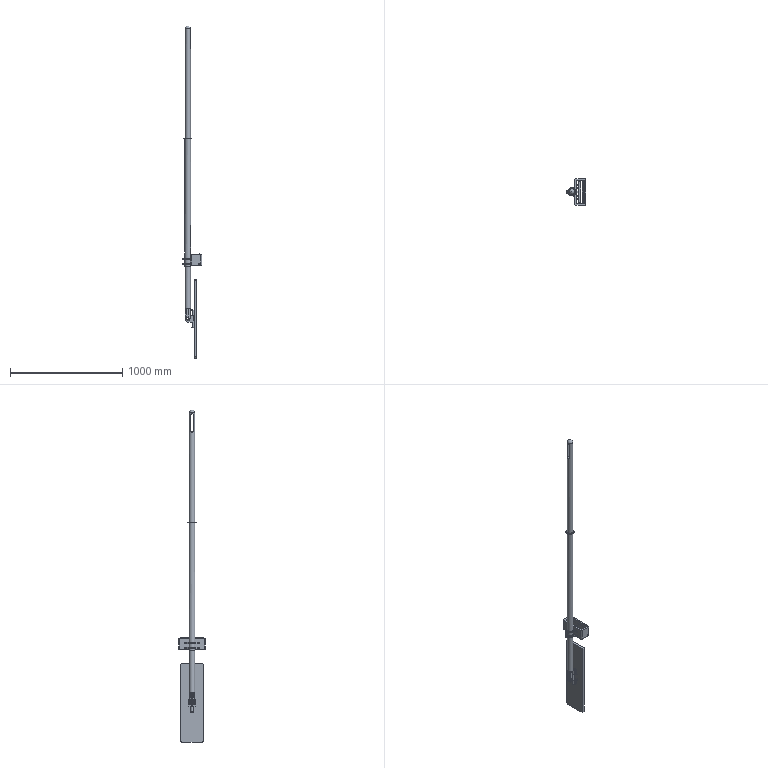Assembly | NX | mm | 5 component files | 5 solids | 280 faces | box 172.52 x 240 x 2960.17 mm | volume 8456671 mm3 | plane 198 | cylinder 68 | spline 8 | torus 4 | sphere 1 | cone 1 | commonest cylinder face diameters 20 x22 10 x13 59.673 x4 8 x4 12 x4 80 x4 22 x3 11 x3
Bill of materials:
unnamed part 1 | 1 |  | Thin rectangular plate with rounded corners and softened edges. Two small protrusions stick out of one face near mid-length.
unnamed part 2 | 1 |  | Long straight shaft with a splined or toothed middle section and a plain cylindrical end section on each side.
unnamed part 3 | 1 |  | Thick block-like lug. One end is a large-radius curve, with a large through-hole near it. A smaller hole runs at right angles through the narrow face.
unnamed part 4 | 1 |  | Very slender straight rod or pin with rounded ends. It has a slot near one end, and the other end looks split or forked.
unnamed part 5 | 1 |  | Tall straight tube with a lip or flange at the top end. Its lower end passes through a ring collar built into an open rectangular box-like frame.
Mates:
1. touch align | model2 1 face | model3 1 face
2. touch align | model2 1 face | model3 1 face
3. touch align | model2 1 face | model1 1 face
4. touch align | model2 1 face | model1 1 face
5. touch align | model4 1 face | model3 1 face
6. touch align | model5 1 face | model4 1 face
7. touch align | model5 1 face | model4 1 face
8. fix | model3 1 component